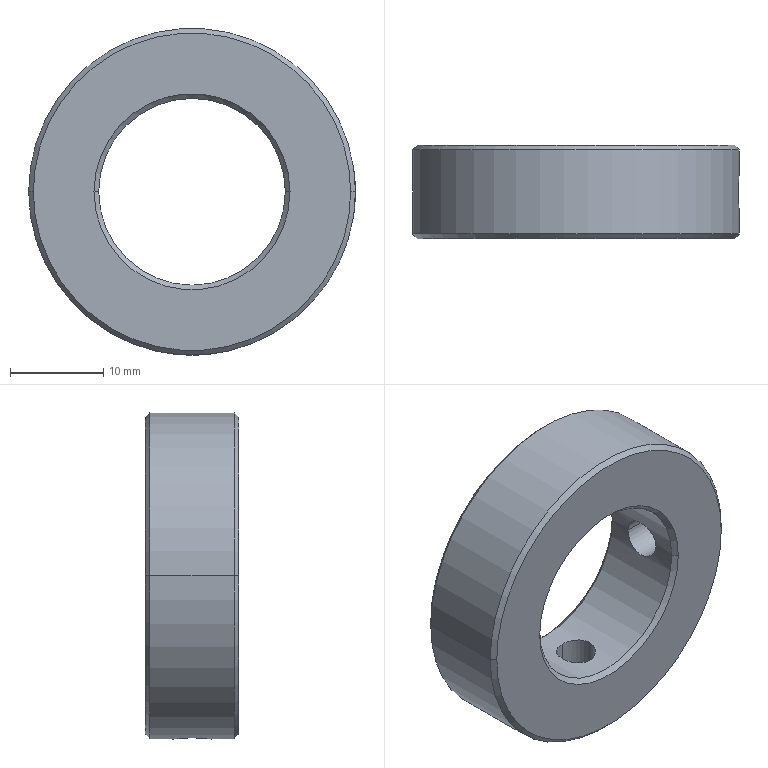Component | SolidWorks | 8TC-A15004-40-23A-1 | 1 solid | 18 faces | box 35 x 10 x 35 mm | volume 6228 mm3 | cone 8 | cylinder 8 | plane 2 | commonest cylinder face diameters 4.2 x4 20 x2 35 x2 | material A3
build123d program:
from build123d import *

# Parameters (mm, degrees)
SKETCH1_R           = 17.5
SKETCH1_R_2         = 10
BOSS_EXTRUDE1_DEPTH = 5
SKETCH2_R           = 2.1
CUT_EXTRUDE1_DEPTH  = 20
CIRPATTERN1_COUNT   = 2
CIRPATTERN1_ANGLE   = 90
CHAMFER1_SIZE       = 0.5


with BuildPart() as part:
    # Sketch1 → Boss-Extrude1 (new, symmetric)
    with BuildSketch(Plane.XY):
        Circle(SKETCH1_R)
        Circle(SKETCH1_R_2, mode=Mode.SUBTRACT)
    extrude(amount=BOSS_EXTRUDE1_DEPTH, both=True)

    # Sketch2 → Cut-Extrude1 (cut)
    with BuildSketch(Plane(origin=(0, 0, 0), x_dir=(1, 0, 0), z_dir=(0, 1, 0))):
        with Locations(Location((0, 0, 0), (0, 0, 270))):
            Circle(SKETCH2_R)
    cut_extrude1 = extrude(amount=-CUT_EXTRUDE1_DEPTH, mode=Mode.SUBTRACT)

    # CirPattern1: Cut-Extrude1 ×2 about axis
    cirpattern1_axis = Axis((0, 0, -5), (0, 0, 1))
    for i in range(1, CIRPATTERN1_COUNT):
        add(cut_extrude1.rotate(cirpattern1_axis, i * CIRPATTERN1_ANGLE / (CIRPATTERN1_COUNT - 1)), mode=Mode.SUBTRACT)

    # Chamfer1
    chamfer1_edges = [part.edges().sort_by_distance(p)[0] for p in [
        (-17.5, 0, -5),
        (-17.5, 0, 5),
        (-10, 0, -5),
        (-10, 0, 5),
    ]]
    chamfer(chamfer1_edges, length=CHAMFER1_SIZE)


solid = part.part

# Placed as in the assembly
solid = solid.moved(Location((40, 212.5, -750), (90, 0, 0)))
STEP:
#1=COLOUR_RGB('',0.7922,0.8196,0.9333);
#2=FILL_AREA_STYLE_COLOUR('',#1);
#3=FILL_AREA_STYLE('',(#2));
#4=SURFACE_STYLE_FILL_AREA(#3);
#5=SURFACE_SIDE_STYLE('',(#4));
#6=SURFACE_STYLE_USAGE(.BOTH.,#5);
#7=PRESENTATION_STYLE_ASSIGNMENT((#6));
#8=CARTESIAN_POINT('',(0.9055,8.563,-29.528));
#9=VERTEX_POINT('',#8);
#10=CARTESIAN_POINT('',(2.244,8.563,-29.528));
#11=VERTEX_POINT('',#10);
#12=CARTESIAN_POINT('',(1.575,8.563,-29.528));
#13=DIRECTION('',(0.,1.,0.));
#14=DIRECTION('',(1.,0.,0.));
#15=AXIS2_PLACEMENT_3D('',#12,#13,#14);
#16=CIRCLE('',#15,0.6693);
#17=EDGE_CURVE('',#9,#11,#16,.T.);
#18=ORIENTED_EDGE('',*,*,#17,.F.);
#19=CARTESIAN_POINT('',(0.8858,8.543,-29.528));
#20=VERTEX_POINT('',#19);
#21=CARTESIAN_POINT('',(0.8858,8.543,-29.528));
#22=DIRECTION('',(-0.7071,-0.7071,0.));
#23=VECTOR('',#22,39.37);
#24=LINE('',#21,#23);
#25=EDGE_CURVE('',#9,#20,#24,.T.);
#26=ORIENTED_EDGE('',*,*,#25,.T.);
#27=CARTESIAN_POINT('',(2.264,8.543,-29.528));
#28=VERTEX_POINT('',#27);
#29=CARTESIAN_POINT('',(1.575,8.543,-29.528));
#30=DIRECTION('',(0.,-1.,0.));
#31=DIRECTION('',(1.,0.,0.));
#32=AXIS2_PLACEMENT_3D('',#29,#30,#31);
#33=CIRCLE('',#32,0.689);
#34=EDGE_CURVE('',#28,#20,#33,.T.);
#35=ORIENTED_EDGE('',*,*,#34,.F.);
#36=CARTESIAN_POINT('',(2.264,8.543,-29.528));
#37=DIRECTION('',(0.7071,-0.7071,0.));
#38=VECTOR('',#37,39.37);
#39=LINE('',#36,#38);
#40=EDGE_CURVE('',#11,#28,#39,.T.);
#41=ORIENTED_EDGE('',*,*,#40,.F.);
#42=EDGE_LOOP('',(#18,#26,#35,#41));
#43=FACE_OUTER_BOUND('',#42,.T.);
#44=CARTESIAN_POINT('',(1.575,8.543,-29.528));
#45=DIRECTION('',(0.,-1.,0.));
#46=DIRECTION('',(1.,0.,0.));
#47=AXIS2_PLACEMENT_3D('',#44,#45,#46);
#48=CONICAL_SURFACE('',#47,0.689,0.7854);
#49=ADVANCED_FACE('',(#43),#48,.T.);
#50=CARTESIAN_POINT('',(1.969,8.543,-29.528));
#51=VERTEX_POINT('',#50);
#52=CARTESIAN_POINT('',(1.181,8.543,-29.528));
#53=VERTEX_POINT('',#52);
#54=CARTESIAN_POINT('',(1.575,8.543,-29.528));
#55=DIRECTION('',(0.,1.,0.));
#56=DIRECTION('',(1.,0.,0.));
#57=AXIS2_PLACEMENT_3D('',#54,#55,#56);
#58=CIRCLE('',#57,0.3937);
#59=EDGE_CURVE('',#51,#53,#58,.T.);
#60=ORIENTED_EDGE('',*,*,#59,.F.);
#61=CARTESIAN_POINT('',(1.988,8.563,-29.528));
#62=VERTEX_POINT('',#61);
#63=CARTESIAN_POINT('',(1.988,8.563,-29.528));
#64=DIRECTION('',(0.7071,0.7071,0.));
#65=VECTOR('',#64,39.37);
#66=LINE('',#63,#65);
#67=EDGE_CURVE('',#51,#62,#66,.T.);
#68=ORIENTED_EDGE('',*,*,#67,.T.);
#69=CARTESIAN_POINT('',(1.161,8.563,-29.528));
#70=VERTEX_POINT('',#69);
#71=CARTESIAN_POINT('',(1.575,8.563,-29.528));
#72=DIRECTION('',(0.,-1.,0.));
#73=DIRECTION('',(1.,0.,0.));
#74=AXIS2_PLACEMENT_3D('',#71,#72,#73);
#75=CIRCLE('',#74,0.4134);
#76=EDGE_CURVE('',#70,#62,#75,.T.);
#77=ORIENTED_EDGE('',*,*,#76,.F.);
#78=CARTESIAN_POINT('',(1.161,8.563,-29.528));
#79=DIRECTION('',(-0.7071,0.7071,0.));
#80=VECTOR('',#79,39.37);
#81=LINE('',#78,#80);
#82=EDGE_CURVE('',#53,#70,#81,.T.);
#83=ORIENTED_EDGE('',*,*,#82,.F.);
#84=EDGE_LOOP('',(#60,#68,#77,#83));
#85=FACE_OUTER_BOUND('',#84,.T.);
#86=CARTESIAN_POINT('',(1.575,8.563,-29.528));
#87=DIRECTION('',(0.,1.,0.));
#88=DIRECTION('',(-1.,0.,0.));
#89=AXIS2_PLACEMENT_3D('',#86,#87,#88);
#90=CONICAL_SURFACE('',#89,0.4134,0.7854);
#91=ADVANCED_FACE('',(#85),#90,.F.);
#92=CARTESIAN_POINT('',(2.244,8.169,-29.528));
#93=VERTEX_POINT('',#92);
#94=CARTESIAN_POINT('',(0.9055,8.169,-29.528));
#95=VERTEX_POINT('',#94);
#96=CARTESIAN_POINT('',(1.575,8.169,-29.528));
#97=DIRECTION('',(0.,-1.,0.));
#98=DIRECTION('',(1.,0.,0.));
#99=AXIS2_PLACEMENT_3D('',#96,#97,#98);
#100=CIRCLE('',#99,0.6693);
#101=EDGE_CURVE('',#93,#95,#100,.T.);
#102=ORIENTED_EDGE('',*,*,#101,.F.);
#103=CARTESIAN_POINT('',(2.264,8.189,-29.528));
#104=VERTEX_POINT('',#103);
#105=CARTESIAN_POINT('',(2.244,8.169,-29.528));
#106=DIRECTION('',(0.7071,0.7071,0.));
#107=VECTOR('',#106,39.37);
#108=LINE('',#105,#107);
#109=EDGE_CURVE('',#93,#104,#108,.T.);
#110=ORIENTED_EDGE('',*,*,#109,.T.);
#111=CARTESIAN_POINT('',(0.8858,8.189,-29.528));
#112=VERTEX_POINT('',#111);
#113=CARTESIAN_POINT('',(1.575,8.189,-29.528));
#114=DIRECTION('',(0.,1.,0.));
#115=DIRECTION('',(1.,0.,0.));
#116=AXIS2_PLACEMENT_3D('',#113,#114,#115);
#117=CIRCLE('',#116,0.689);
#118=EDGE_CURVE('',#112,#104,#117,.T.);
#119=ORIENTED_EDGE('',*,*,#118,.F.);
#120=CARTESIAN_POINT('',(0.9055,8.169,-29.528));
#121=DIRECTION('',(-0.7071,0.7071,0.));
#122=VECTOR('',#121,39.37);
#123=LINE('',#120,#122);
#124=EDGE_CURVE('',#95,#112,#123,.T.);
#125=ORIENTED_EDGE('',*,*,#124,.F.);
#126=EDGE_LOOP('',(#102,#110,#119,#125));
#127=FACE_OUTER_BOUND('',#126,.T.);
#128=CARTESIAN_POINT('',(1.575,8.169,-29.528));
#129=DIRECTION('',(0.,1.,0.));
#130=DIRECTION('',(-1.,0.,0.));
#131=AXIS2_PLACEMENT_3D('',#128,#129,#130);
#132=CONICAL_SURFACE('',#131,0.6693,0.7854);
#133=ADVANCED_FACE('',(#127),#132,.T.);
#134=CARTESIAN_POINT('',(1.181,8.189,-29.528));
#135=VERTEX_POINT('',#134);
#136=CARTESIAN_POINT('',(1.969,8.189,-29.528));
#137=VERTEX_POINT('',#136);
#138=CARTESIAN_POINT('',(1.575,8.189,-29.528));
#139=DIRECTION('',(0.,-1.,0.));
#140=DIRECTION('',(1.,0.,0.));
#141=AXIS2_PLACEMENT_3D('',#138,#139,#140);
#142=CIRCLE('',#141,0.3937);
#143=EDGE_CURVE('',#135,#137,#142,.T.);
#144=ORIENTED_EDGE('',*,*,#143,.F.);
#145=CARTESIAN_POINT('',(1.161,8.169,-29.528));
#146=VERTEX_POINT('',#145);
#147=CARTESIAN_POINT('',(1.181,8.189,-29.528));
#148=DIRECTION('',(-0.7071,-0.7071,0.));
#149=VECTOR('',#148,39.37);
#150=LINE('',#147,#149);
#151=EDGE_CURVE('',#135,#146,#150,.T.);
#152=ORIENTED_EDGE('',*,*,#151,.T.);
#153=CARTESIAN_POINT('',(1.988,8.169,-29.528));
#154=VERTEX_POINT('',#153);
#155=CARTESIAN_POINT('',(1.575,8.169,-29.528));
#156=DIRECTION('',(0.,1.,0.));
#157=DIRECTION('',(1.,0.,0.));
#158=AXIS2_PLACEMENT_3D('',#155,#156,#157);
#159=CIRCLE('',#158,0.4134);
#160=EDGE_CURVE('',#154,#146,#159,.T.);
#161=ORIENTED_EDGE('',*,*,#160,.F.);
#162=CARTESIAN_POINT('',(1.969,8.189,-29.528));
#163=DIRECTION('',(0.7071,-0.7071,0.));
#164=VECTOR('',#163,39.37);
#165=LINE('',#162,#164);
#166=EDGE_CURVE('',#137,#154,#165,.T.);
#167=ORIENTED_EDGE('',*,*,#166,.F.);
#168=EDGE_LOOP('',(#144,#152,#161,#167));
#169=FACE_OUTER_BOUND('',#168,.T.);
#170=CARTESIAN_POINT('',(1.575,8.189,-29.528));
#171=DIRECTION('',(0.,-1.,0.));
#172=DIRECTION('',(1.,0.,0.));
#173=AXIS2_PLACEMENT_3D('',#170,#171,#172);
#174=CONICAL_SURFACE('',#173,0.3937,0.7854);
#175=ADVANCED_FACE('',(#169),#174,.F.);
#176=CARTESIAN_POINT('',(2.264,8.449,-29.528));
#177=VERTEX_POINT('',#176);
#178=CARTESIAN_POINT('',(2.264,8.283,-29.528));
#179=VERTEX_POINT('',#178);
#180=CARTESIAN_POINT('',(2.264,8.449,-29.528));
#181=CARTESIAN_POINT('',(2.264,8.449,-29.538));
#182=CARTESIAN_POINT('',(2.264,8.447,-29.549));
#183=CARTESIAN_POINT('',(2.263,8.438,-29.569));
#184=CARTESIAN_POINT('',(2.262,8.432,-29.578));
#185=CARTESIAN_POINT('',(2.261,8.421,-29.59));
#186=CARTESIAN_POINT('',(2.261,8.417,-29.593));
#187=CARTESIAN_POINT('',(2.26,8.408,-29.599));
#188=CARTESIAN_POINT('',(2.26,8.403,-29.602));
#189=CARTESIAN_POINT('',(2.259,8.393,-29.606));
#190=CARTESIAN_POINT('',(2.259,8.388,-29.608));
#191=CARTESIAN_POINT('',(2.259,8.377,-29.61));
#192=CARTESIAN_POINT('',(2.259,8.372,-29.61));
#193=CARTESIAN_POINT('',(2.259,8.361,-29.61));
#194=CARTESIAN_POINT('',(2.259,8.355,-29.61));
#195=CARTESIAN_POINT('',(2.259,8.345,-29.608));
#196=CARTESIAN_POINT('',(2.259,8.34,-29.606));
#197=CARTESIAN_POINT('',(2.26,8.33,-29.602));
#198=CARTESIAN_POINT('',(2.26,8.325,-29.599));
#199=CARTESIAN_POINT('',(2.261,8.316,-29.593));
#200=CARTESIAN_POINT('',(2.261,8.312,-29.59));
#201=CARTESIAN_POINT('',(2.262,8.3,-29.578));
#202=CARTESIAN_POINT('',(2.263,8.294,-29.569));
#203=CARTESIAN_POINT('',(2.264,8.286,-29.549));
#204=CARTESIAN_POINT('',(2.264,8.283,-29.538));
#205=CARTESIAN_POINT('',(2.264,8.283,-29.528));
#206=B_SPLINE_CURVE_WITH_KNOTS('',3,(#180,#181,#182,#183,#184,#185,#186,#187,#188,#189,#190,#191,#192,#193,#194,#195,#196,#197,#198,#199,#200,#201,#202,#203,#204,#205),.UNSPECIFIED.,.F.,.F.,(4,2,2,2,2,2,2,2,2,2,2,2,4),(0.006571,0.007393,0.008214,0.008625,0.009035,0.009446,0.009856,0.01027,0.01068,0.01109,0.0115,0.01232,0.01314),.UNSPECIFIED.);
#207=EDGE_CURVE('',#177,#179,#206,.T.);
#208=ORIENTED_EDGE('',*,*,#207,.F.);
#209=CARTESIAN_POINT('',(1.969,8.449,-29.528));
#210=VERTEX_POINT('',#209);
#211=CARTESIAN_POINT('',(2.362,8.449,-29.528));
#212=DIRECTION('',(-1.,0.,-0.));
#213=VECTOR('',#212,39.37);
#214=LINE('',#211,#213);
#215=EDGE_CURVE('',#177,#210,#214,.T.);
#216=ORIENTED_EDGE('',*,*,#215,.T.);
#217=CARTESIAN_POINT('',(1.969,8.283,-29.528));
#218=VERTEX_POINT('',#217);
#219=CARTESIAN_POINT('',(1.969,8.449,-29.528));
#220=CARTESIAN_POINT('',(1.969,8.449,-29.538));
#221=CARTESIAN_POINT('',(1.968,8.447,-29.549));
#222=CARTESIAN_POINT('',(1.967,8.44,-29.564));
#223=CARTESIAN_POINT('',(1.966,8.438,-29.569));
#224=CARTESIAN_POINT('',(1.965,8.432,-29.578));
#225=CARTESIAN_POINT('',(1.965,8.428,-29.582));
#226=CARTESIAN_POINT('',(1.964,8.421,-29.59));
#227=CARTESIAN_POINT('',(1.963,8.417,-29.593));
#228=CARTESIAN_POINT('',(1.962,8.408,-29.599));
#229=CARTESIAN_POINT('',(1.961,8.403,-29.602));
#230=CARTESIAN_POINT('',(1.96,8.388,-29.608));
#231=CARTESIAN_POINT('',(1.96,8.377,-29.61));
#232=CARTESIAN_POINT('',(1.96,8.361,-29.61));
#233=CARTESIAN_POINT('',(1.96,8.355,-29.61));
#234=CARTESIAN_POINT('',(1.96,8.345,-29.608));
#235=CARTESIAN_POINT('',(1.961,8.339,-29.606));
#236=CARTESIAN_POINT('',(1.961,8.329,-29.602));
#237=CARTESIAN_POINT('',(1.962,8.325,-29.599));
#238=CARTESIAN_POINT('',(1.963,8.316,-29.593));
#239=CARTESIAN_POINT('',(1.964,8.312,-29.59));
#240=CARTESIAN_POINT('',(1.965,8.3,-29.578));
#241=CARTESIAN_POINT('',(1.966,8.294,-29.569));
#242=CARTESIAN_POINT('',(1.968,8.288,-29.554));
#243=CARTESIAN_POINT('',(1.968,8.286,-29.549));
#244=CARTESIAN_POINT('',(1.968,8.284,-29.538));
#245=CARTESIAN_POINT('',(1.969,8.283,-29.533));
#246=CARTESIAN_POINT('',(1.969,8.283,-29.528));
#247=B_SPLINE_CURVE_WITH_KNOTS('',3,(#219,#220,#221,#222,#223,#224,#225,#226,#227,#228,#229,#230,#231,#232,#233,#234,#235,#236,#237,#238,#239,#240,#241,#242,#243,#244,#245,#246),.UNSPECIFIED.,.F.,.F.,(4,2,2,2,2,2,2,2,2,2,2,2,2,4),(0.006584,0.007407,0.007818,0.008229,0.008641,0.009052,0.009875,0.01029,0.0107,0.01111,0.01152,0.01234,0.01275,0.01317),.UNSPECIFIED.);
#248=EDGE_CURVE('',#210,#218,#247,.T.);
#249=ORIENTED_EDGE('',*,*,#248,.T.);
#250=CARTESIAN_POINT('',(2.362,8.283,-29.528));
#251=DIRECTION('',(-1.,0.,-0.));
#252=VECTOR('',#251,39.37);
#253=LINE('',#250,#252);
#254=EDGE_CURVE('',#179,#218,#253,.T.);
#255=ORIENTED_EDGE('',*,*,#254,.F.);
#256=EDGE_LOOP('',(#208,#216,#249,#255));
#257=FACE_OUTER_BOUND('',#256,.T.);
#258=CARTESIAN_POINT('',(2.362,8.366,-29.528));
#259=DIRECTION('',(-1.,0.,-0.));
#260=DIRECTION('',(0.,-1.,0.));
#261=AXIS2_PLACEMENT_3D('',#258,#259,#260);
#262=CYLINDRICAL_SURFACE('',#261,0.08268);
#263=ADVANCED_FACE('',(#257),#262,.F.);
#264=CARTESIAN_POINT('',(1.575,8.449,-30.217));
#265=VERTEX_POINT('',#264);
#266=CARTESIAN_POINT('',(1.575,8.283,-30.217));
#267=VERTEX_POINT('',#266);
#268=CARTESIAN_POINT('',(1.575,8.449,-30.217));
#269=CARTESIAN_POINT('',(1.564,8.449,-30.217));
#270=CARTESIAN_POINT('',(1.553,8.447,-30.216));
#271=CARTESIAN_POINT('',(1.533,8.438,-30.215));
#272=CARTESIAN_POINT('',(1.524,8.432,-30.215));
#273=CARTESIAN_POINT('',(1.513,8.421,-30.214));
#274=CARTESIAN_POINT('',(1.509,8.417,-30.213));
#275=CARTESIAN_POINT('',(1.503,8.408,-30.213));
#276=CARTESIAN_POINT('',(1.501,8.403,-30.213));
#277=CARTESIAN_POINT('',(1.496,8.393,-30.212));
#278=CARTESIAN_POINT('',(1.495,8.388,-30.212));
#279=CARTESIAN_POINT('',(1.493,8.377,-30.212));
#280=CARTESIAN_POINT('',(1.492,8.372,-30.212));
#281=CARTESIAN_POINT('',(1.492,8.361,-30.212));
#282=CARTESIAN_POINT('',(1.493,8.355,-30.212));
#283=CARTESIAN_POINT('',(1.495,8.345,-30.212));
#284=CARTESIAN_POINT('',(1.496,8.34,-30.212));
#285=CARTESIAN_POINT('',(1.5,8.33,-30.213));
#286=CARTESIAN_POINT('',(1.503,8.325,-30.213));
#287=CARTESIAN_POINT('',(1.509,8.316,-30.213));
#288=CARTESIAN_POINT('',(1.512,8.312,-30.214));
#289=CARTESIAN_POINT('',(1.524,8.3,-30.215));
#290=CARTESIAN_POINT('',(1.533,8.294,-30.215));
#291=CARTESIAN_POINT('',(1.553,8.286,-30.216));
#292=CARTESIAN_POINT('',(1.564,8.283,-30.217));
#293=CARTESIAN_POINT('',(1.575,8.283,-30.217));
#294=B_SPLINE_CURVE_WITH_KNOTS('',3,(#268,#269,#270,#271,#272,#273,#274,#275,#276,#277,#278,#279,#280,#281,#282,#283,#284,#285,#286,#287,#288,#289,#290,#291,#292,#293),.UNSPECIFIED.,.F.,.F.,(4,2,2,2,2,2,2,2,2,2,2,2,4),(0.006571,0.007393,0.008214,0.008625,0.009035,0.009446,0.009856,0.01027,0.01068,0.01109,0.0115,0.01232,0.01314),.UNSPECIFIED.);
#295=EDGE_CURVE('',#265,#267,#294,.T.);
#296=ORIENTED_EDGE('',*,*,#295,.F.);
#297=CARTESIAN_POINT('',(1.575,8.449,-29.921));
#298=VERTEX_POINT('',#297);
#299=CARTESIAN_POINT('',(1.575,8.449,-30.315));
#300=DIRECTION('',(0.,0.,1.));
#301=VECTOR('',#300,39.37);
#302=LINE('',#299,#301);
#303=EDGE_CURVE('',#265,#298,#302,.T.);
#304=ORIENTED_EDGE('',*,*,#303,.T.);
#305=CARTESIAN_POINT('',(1.575,8.283,-29.921));
#306=VERTEX_POINT('',#305);
#307=CARTESIAN_POINT('',(1.575,8.449,-29.921));
#308=CARTESIAN_POINT('',(1.564,8.449,-29.921));
#309=CARTESIAN_POINT('',(1.553,8.447,-29.921));
#310=CARTESIAN_POINT('',(1.538,8.44,-29.92));
#311=CARTESIAN_POINT('',(1.533,8.438,-29.919));
#312=CARTESIAN_POINT('',(1.524,8.432,-29.918));
#313=CARTESIAN_POINT('',(1.52,8.428,-29.917));
#314=CARTESIAN_POINT('',(1.513,8.421,-29.916));
#315=CARTESIAN_POINT('',(1.509,8.417,-29.916));
#316=CARTESIAN_POINT('',(1.503,8.408,-29.915));
#317=CARTESIAN_POINT('',(1.501,8.403,-29.914));
#318=CARTESIAN_POINT('',(1.494,8.388,-29.913));
#319=CARTESIAN_POINT('',(1.492,8.377,-29.912));
#320=CARTESIAN_POINT('',(1.492,8.361,-29.912));
#321=CARTESIAN_POINT('',(1.493,8.355,-29.913));
#322=CARTESIAN_POINT('',(1.495,8.345,-29.913));
#323=CARTESIAN_POINT('',(1.496,8.339,-29.913));
#324=CARTESIAN_POINT('',(1.5,8.329,-29.914));
#325=CARTESIAN_POINT('',(1.503,8.325,-29.915));
#326=CARTESIAN_POINT('',(1.509,8.316,-29.916));
#327=CARTESIAN_POINT('',(1.513,8.312,-29.916));
#328=CARTESIAN_POINT('',(1.524,8.3,-29.918));
#329=CARTESIAN_POINT('',(1.533,8.294,-29.919));
#330=CARTESIAN_POINT('',(1.548,8.288,-29.92));
#331=CARTESIAN_POINT('',(1.553,8.286,-29.921));
#332=CARTESIAN_POINT('',(1.564,8.284,-29.921));
#333=CARTESIAN_POINT('',(1.569,8.283,-29.921));
#334=CARTESIAN_POINT('',(1.575,8.283,-29.921));
#335=B_SPLINE_CURVE_WITH_KNOTS('',3,(#307,#308,#309,#310,#311,#312,#313,#314,#315,#316,#317,#318,#319,#320,#321,#322,#323,#324,#325,#326,#327,#328,#329,#330,#331,#332,#333,#334),.UNSPECIFIED.,.F.,.F.,(4,2,2,2,2,2,2,2,2,2,2,2,2,4),(0.006584,0.007407,0.007818,0.008229,0.008641,0.009052,0.009875,0.01029,0.0107,0.01111,0.01152,0.01234,0.01275,0.01317),.UNSPECIFIED.);
#336=EDGE_CURVE('',#298,#306,#335,.T.);
#337=ORIENTED_EDGE('',*,*,#336,.T.);
#338=CARTESIAN_POINT('',(1.575,8.283,-30.315));
#339=DIRECTION('',(0.,0.,1.));
#340=VECTOR('',#339,39.37);
#341=LINE('',#338,#340);
#342=EDGE_CURVE('',#267,#306,#341,.T.);
#343=ORIENTED_EDGE('',*,*,#342,.F.);
#344=EDGE_LOOP('',(#296,#304,#337,#343));
#345=FACE_OUTER_BOUND('',#344,.T.);
#346=CARTESIAN_POINT('',(1.575,8.366,-30.315));
#347=DIRECTION('',(0.,0.,1.));
#348=DIRECTION('',(0.,-1.,0.));
#349=AXIS2_PLACEMENT_3D('',#346,#347,#348);
#350=CYLINDRICAL_SURFACE('',#349,0.08268);
#351=ADVANCED_FACE('',(#345),#350,.F.);
#352=CARTESIAN_POINT('',(1.575,8.283,-29.921));
#353=CARTESIAN_POINT('',(1.58,8.283,-29.921));
#354=CARTESIAN_POINT('',(1.586,8.284,-29.921));
#355=CARTESIAN_POINT('',(1.596,8.286,-29.921));
#356=CARTESIAN_POINT('',(1.602,8.288,-29.92));
#357=CARTESIAN_POINT('',(1.612,8.292,-29.92));
#358=CARTESIAN_POINT('',(1.616,8.294,-29.919));
#359=CARTESIAN_POINT('',(1.625,8.3,-29.918));
#360=CARTESIAN_POINT('',(1.629,8.304,-29.917));
#361=CARTESIAN_POINT('',(1.641,8.315,-29.916));
#362=CARTESIAN_POINT('',(1.647,8.325,-29.915));
#363=CARTESIAN_POINT('',(1.653,8.339,-29.913));
#364=CARTESIAN_POINT('',(1.655,8.345,-29.913));
#365=CARTESIAN_POINT('',(1.657,8.355,-29.913));
#366=CARTESIAN_POINT('',(1.657,8.361,-29.912));
#367=CARTESIAN_POINT('',(1.657,8.372,-29.912));
#368=CARTESIAN_POINT('',(1.657,8.377,-29.913));
#369=CARTESIAN_POINT('',(1.655,8.388,-29.913));
#370=CARTESIAN_POINT('',(1.653,8.393,-29.913));
#371=CARTESIAN_POINT('',(1.647,8.408,-29.915));
#372=CARTESIAN_POINT('',(1.641,8.417,-29.916));
#373=CARTESIAN_POINT('',(1.629,8.428,-29.917));
#374=CARTESIAN_POINT('',(1.625,8.432,-29.918));
#375=CARTESIAN_POINT('',(1.616,8.438,-29.919));
#376=CARTESIAN_POINT('',(1.611,8.44,-29.92));
#377=CARTESIAN_POINT('',(1.601,8.445,-29.92));
#378=CARTESIAN_POINT('',(1.596,8.446,-29.921));
#379=CARTESIAN_POINT('',(1.586,8.448,-29.921));
#380=CARTESIAN_POINT('',(1.58,8.449,-29.921));
#381=CARTESIAN_POINT('',(1.575,8.449,-29.921));
#382=B_SPLINE_CURVE_WITH_KNOTS('',3,(#352,#353,#354,#355,#356,#357,#358,#359,#360,#361,#362,#363,#364,#365,#366,#367,#368,#369,#370,#371,#372,#373,#374,#375,#376,#377,#378,#379,#380,#381),.UNSPECIFIED.,.F.,.F.,(4,2,2,2,2,2,2,2,2,2,2,2,2,2,4),(0.,0.0004115,0.000823,0.001234,0.001646,0.002469,0.00288,0.003292,0.003703,0.004115,0.004938,0.005349,0.005761,0.006172,0.006584),.UNSPECIFIED.);
#383=EDGE_CURVE('',#306,#298,#382,.T.);
#384=ORIENTED_EDGE('',*,*,#383,.F.);
#385=ORIENTED_EDGE('',*,*,#336,.F.);
#386=EDGE_LOOP('',(#384,#385));
#387=FACE_BOUND('',#386,.T.);
#388=ORIENTED_EDGE('',*,*,#143,.T.);
#389=CARTESIAN_POINT('',(1.969,8.169,-29.528));
#390=DIRECTION('',(0.,1.,0.));
#391=VECTOR('',#390,39.37);
#392=LINE('',#389,#391);
#393=EDGE_CURVE('',#137,#218,#392,.T.);
#394=ORIENTED_EDGE('',*,*,#393,.T.);
#395=ORIENTED_EDGE('',*,*,#248,.F.);
#396=CARTESIAN_POINT('',(1.969,8.169,-29.528));
#397=DIRECTION('',(0.,1.,0.));
#398=VECTOR('',#397,39.37);
#399=LINE('',#396,#398);
#400=EDGE_CURVE('',#210,#51,#399,.T.);
#401=ORIENTED_EDGE('',*,*,#400,.T.);
#402=ORIENTED_EDGE('',*,*,#59,.T.);
#403=CARTESIAN_POINT('',(1.181,8.169,-29.528));
#404=DIRECTION('',(0.,1.,0.));
#405=VECTOR('',#404,39.37);
#406=LINE('',#403,#405);
#407=EDGE_CURVE('',#135,#53,#406,.T.);
#408=ORIENTED_EDGE('',*,*,#407,.F.);
#409=EDGE_LOOP('',(#388,#394,#395,#401,#402,#408));
#410=FACE_OUTER_BOUND('',#409,.T.);
#411=CARTESIAN_POINT('',(1.575,8.169,-29.528));
#412=DIRECTION('',(0.,1.,0.));
#413=DIRECTION('',(-1.,0.,0.));
#414=AXIS2_PLACEMENT_3D('',#411,#412,#413);
#415=CYLINDRICAL_SURFACE('',#414,0.3937);
#416=ADVANCED_FACE('',(#387,#410),#415,.F.);
#417=ORIENTED_EDGE('',*,*,#118,.T.);
#418=CARTESIAN_POINT('',(2.264,8.169,-29.528));
#419=DIRECTION('',(0.,1.,0.));
#420=VECTOR('',#419,39.37);
#421=LINE('',#418,#420);
#422=EDGE_CURVE('',#104,#179,#421,.T.);
#423=ORIENTED_EDGE('',*,*,#422,.T.);
#424=CARTESIAN_POINT('',(2.264,8.283,-29.528));
#425=CARTESIAN_POINT('',(2.264,8.283,-29.522));
#426=CARTESIAN_POINT('',(2.264,8.284,-29.517));
#427=CARTESIAN_POINT('',(2.263,8.286,-29.506));
#428=CARTESIAN_POINT('',(2.263,8.288,-29.501));
#429=CARTESIAN_POINT('',(2.263,8.292,-29.491));
#430=CARTESIAN_POINT('',(2.263,8.294,-29.486));
#431=CARTESIAN_POINT('',(2.262,8.3,-29.477));
#432=CARTESIAN_POINT('',(2.262,8.304,-29.473));
#433=CARTESIAN_POINT('',(2.261,8.315,-29.461));
#434=CARTESIAN_POINT('',(2.26,8.325,-29.455));
#435=CARTESIAN_POINT('',(2.259,8.344,-29.447));
#436=CARTESIAN_POINT('',(2.259,8.355,-29.445));
#437=CARTESIAN_POINT('',(2.259,8.372,-29.445));
#438=CARTESIAN_POINT('',(2.259,8.377,-29.445));
#439=CARTESIAN_POINT('',(2.259,8.388,-29.448));
#440=CARTESIAN_POINT('',(2.259,8.393,-29.449));
#441=CARTESIAN_POINT('',(2.26,8.403,-29.453));
#442=CARTESIAN_POINT('',(2.26,8.408,-29.456));
#443=CARTESIAN_POINT('',(2.261,8.417,-29.462));
#444=CARTESIAN_POINT('',(2.261,8.421,-29.465));
#445=CARTESIAN_POINT('',(2.262,8.428,-29.473));
#446=CARTESIAN_POINT('',(2.262,8.432,-29.477));
#447=CARTESIAN_POINT('',(2.263,8.438,-29.486));
#448=CARTESIAN_POINT('',(2.263,8.44,-29.491));
#449=CARTESIAN_POINT('',(2.263,8.445,-29.501));
#450=CARTESIAN_POINT('',(2.263,8.446,-29.506));
#451=CARTESIAN_POINT('',(2.264,8.448,-29.517));
#452=CARTESIAN_POINT('',(2.264,8.449,-29.522));
#453=CARTESIAN_POINT('',(2.264,8.449,-29.528));
#454=B_SPLINE_CURVE_WITH_KNOTS('',3,(#424,#425,#426,#427,#428,#429,#430,#431,#432,#433,#434,#435,#436,#437,#438,#439,#440,#441,#442,#443,#444,#445,#446,#447,#448,#449,#450,#451,#452,#453),.UNSPECIFIED.,.F.,.F.,(4,2,2,2,2,2,2,2,2,2,2,2,2,2,4),(0.,0.0004107,0.0008214,0.001232,0.001643,0.002464,0.003286,0.003696,0.004107,0.004518,0.004929,0.005339,0.00575,0.006161,0.006571),.UNSPECIFIED.);
#455=EDGE_CURVE('',#179,#177,#454,.T.);
#456=ORIENTED_EDGE('',*,*,#455,.T.);
#457=CARTESIAN_POINT('',(2.264,8.169,-29.528));
#458=DIRECTION('',(0.,1.,0.));
#459=VECTOR('',#458,39.37);
#460=LINE('',#457,#459);
#461=EDGE_CURVE('',#177,#28,#460,.T.);
#462=ORIENTED_EDGE('',*,*,#461,.T.);
#463=ORIENTED_EDGE('',*,*,#34,.T.);
#464=CARTESIAN_POINT('',(0.8858,8.169,-29.528));
#465=DIRECTION('',(0.,1.,0.));
#466=VECTOR('',#465,39.37);
#467=LINE('',#464,#466);
#468=EDGE_CURVE('',#112,#20,#467,.T.);
#469=ORIENTED_EDGE('',*,*,#468,.F.);
#470=EDGE_LOOP('',(#417,#423,#456,#462,#463,#469));
#471=FACE_OUTER_BOUND('',#470,.T.);
#472=CARTESIAN_POINT('',(1.575,8.169,-29.528));
#473=DIRECTION('',(0.,1.,0.));
#474=DIRECTION('',(-1.,0.,0.));
#475=AXIS2_PLACEMENT_3D('',#472,#473,#474);
#476=CYLINDRICAL_SURFACE('',#475,0.689);
#477=ADVANCED_FACE('',(#471),#476,.T.);
#478=ORIENTED_EDGE('',*,*,#160,.T.);
#479=CARTESIAN_POINT('',(1.575,8.169,-29.528));
#480=DIRECTION('',(0.,1.,0.));
#481=DIRECTION('',(1.,0.,0.));
#482=AXIS2_PLACEMENT_3D('',#479,#480,#481);
#483=CIRCLE('',#482,0.4134);
#484=EDGE_CURVE('',#146,#154,#483,.T.);
#485=ORIENTED_EDGE('',*,*,#484,.T.);
#486=EDGE_LOOP('',(#478,#485));
#487=FACE_BOUND('',#486,.T.);
#488=CARTESIAN_POINT('',(1.575,8.169,-29.528));
#489=DIRECTION('',(0.,-1.,0.));
#490=DIRECTION('',(1.,0.,0.));
#491=AXIS2_PLACEMENT_3D('',#488,#489,#490);
#492=CIRCLE('',#491,0.6693);
#493=EDGE_CURVE('',#95,#93,#492,.T.);
#494=ORIENTED_EDGE('',*,*,#493,.T.);
#495=ORIENTED_EDGE('',*,*,#101,.T.);
#496=EDGE_LOOP('',(#494,#495));
#497=FACE_OUTER_BOUND('',#496,.T.);
#498=CARTESIAN_POINT('',(1.575,8.169,-29.528));
#499=DIRECTION('',(0.,-1.,0.));
#500=DIRECTION('',(1.,0.,0.));
#501=AXIS2_PLACEMENT_3D('',#498,#499,#500);
#502=PLANE('',#501);
#503=ADVANCED_FACE('',(#487,#497),#502,.T.);
#504=ORIENTED_EDGE('',*,*,#76,.T.);
#505=CARTESIAN_POINT('',(1.575,8.563,-29.528));
#506=DIRECTION('',(0.,-1.,0.));
#507=DIRECTION('',(1.,0.,0.));
#508=AXIS2_PLACEMENT_3D('',#505,#506,#507);
#509=CIRCLE('',#508,0.4134);
#510=EDGE_CURVE('',#62,#70,#509,.T.);
#511=ORIENTED_EDGE('',*,*,#510,.T.);
#512=EDGE_LOOP('',(#504,#511));
#513=FACE_BOUND('',#512,.T.);
#514=CARTESIAN_POINT('',(1.575,8.563,-29.528));
#515=DIRECTION('',(0.,1.,0.));
#516=DIRECTION('',(1.,0.,0.));
#517=AXIS2_PLACEMENT_3D('',#514,#515,#516);
#518=CIRCLE('',#517,0.6693);
#519=EDGE_CURVE('',#11,#9,#518,.T.);
#520=ORIENTED_EDGE('',*,*,#519,.T.);
#521=ORIENTED_EDGE('',*,*,#17,.T.);
#522=EDGE_LOOP('',(#520,#521));
#523=FACE_OUTER_BOUND('',#522,.T.);
#524=CARTESIAN_POINT('',(1.575,8.563,-29.528));
#525=DIRECTION('',(0.,-1.,0.));
#526=DIRECTION('',(1.,0.,0.));
#527=AXIS2_PLACEMENT_3D('',#524,#525,#526);
#528=PLANE('',#527);
#529=ADVANCED_FACE('',(#513,#523),#528,.F.);
#530=ORIENTED_EDGE('',*,*,#422,.F.);
#531=CARTESIAN_POINT('',(1.575,8.189,-29.528));
#532=DIRECTION('',(0.,1.,0.));
#533=DIRECTION('',(1.,0.,0.));
#534=AXIS2_PLACEMENT_3D('',#531,#532,#533);
#535=CIRCLE('',#534,0.689);
#536=EDGE_CURVE('',#104,#112,#535,.T.);
#537=ORIENTED_EDGE('',*,*,#536,.T.);
#538=ORIENTED_EDGE('',*,*,#468,.T.);
#539=CARTESIAN_POINT('',(1.575,8.543,-29.528));
#540=DIRECTION('',(0.,-1.,0.));
#541=DIRECTION('',(1.,0.,0.));
#542=AXIS2_PLACEMENT_3D('',#539,#540,#541);
#543=CIRCLE('',#542,0.689);
#544=EDGE_CURVE('',#20,#28,#543,.T.);
#545=ORIENTED_EDGE('',*,*,#544,.T.);
#546=ORIENTED_EDGE('',*,*,#461,.F.);
#547=ORIENTED_EDGE('',*,*,#207,.T.);
#548=EDGE_LOOP('',(#530,#537,#538,#545,#546,#547));
#549=FACE_OUTER_BOUND('',#548,.T.);
#550=CARTESIAN_POINT('',(1.575,8.283,-30.217));
#551=CARTESIAN_POINT('',(1.58,8.283,-30.217));
#552=CARTESIAN_POINT('',(1.586,8.284,-30.216));
#553=CARTESIAN_POINT('',(1.596,8.286,-30.216));
#554=CARTESIAN_POINT('',(1.601,8.288,-30.216));
#555=CARTESIAN_POINT('',(1.611,8.292,-30.216));
#556=CARTESIAN_POINT('',(1.616,8.294,-30.215));
#557=CARTESIAN_POINT('',(1.625,8.3,-30.215));
#558=CARTESIAN_POINT('',(1.629,8.304,-30.214));
#559=CARTESIAN_POINT('',(1.641,8.315,-30.213));
#560=CARTESIAN_POINT('',(1.647,8.325,-30.213));
#561=CARTESIAN_POINT('',(1.655,8.344,-30.212));
#562=CARTESIAN_POINT('',(1.657,8.355,-30.212));
#563=CARTESIAN_POINT('',(1.657,8.372,-30.212));
#564=CARTESIAN_POINT('',(1.657,8.377,-30.212));
#565=CARTESIAN_POINT('',(1.655,8.388,-30.212));
#566=CARTESIAN_POINT('',(1.653,8.393,-30.212));
#567=CARTESIAN_POINT('',(1.649,8.403,-30.213));
#568=CARTESIAN_POINT('',(1.647,8.408,-30.213));
#569=CARTESIAN_POINT('',(1.641,8.417,-30.213));
#570=CARTESIAN_POINT('',(1.637,8.421,-30.214));
#571=CARTESIAN_POINT('',(1.629,8.428,-30.214));
#572=CARTESIAN_POINT('',(1.625,8.432,-30.215));
#573=CARTESIAN_POINT('',(1.616,8.438,-30.215));
#574=CARTESIAN_POINT('',(1.611,8.44,-30.216));
#575=CARTESIAN_POINT('',(1.601,8.445,-30.216));
#576=CARTESIAN_POINT('',(1.596,8.446,-30.216));
#577=CARTESIAN_POINT('',(1.586,8.448,-30.216));
#578=CARTESIAN_POINT('',(1.58,8.449,-30.217));
#579=CARTESIAN_POINT('',(1.575,8.449,-30.217));
#580=B_SPLINE_CURVE_WITH_KNOTS('',3,(#550,#551,#552,#553,#554,#555,#556,#557,#558,#559,#560,#561,#562,#563,#564,#565,#566,#567,#568,#569,#570,#571,#572,#573,#574,#575,#576,#577,#578,#579),.UNSPECIFIED.,.F.,.F.,(4,2,2,2,2,2,2,2,2,2,2,2,2,2,4),(0.,0.0004107,0.0008214,0.001232,0.001643,0.002464,0.003286,0.003696,0.004107,0.004518,0.004929,0.005339,0.00575,0.006161,0.006571),.UNSPECIFIED.);
#581=EDGE_CURVE('',#267,#265,#580,.T.);
#582=ORIENTED_EDGE('',*,*,#581,.T.);
#583=ORIENTED_EDGE('',*,*,#295,.T.);
#584=EDGE_LOOP('',(#582,#583));
#585=FACE_BOUND('',#584,.T.);
#586=CARTESIAN_POINT('',(1.575,8.169,-29.528));
#587=DIRECTION('',(0.,1.,0.));
#588=DIRECTION('',(-1.,0.,0.));
#589=AXIS2_PLACEMENT_3D('',#586,#587,#588);
#590=CYLINDRICAL_SURFACE('',#589,0.689);
#591=ADVANCED_FACE('',(#549,#585),#590,.T.);
#592=ORIENTED_EDGE('',*,*,#393,.F.);
#593=CARTESIAN_POINT('',(1.575,8.189,-29.528));
#594=DIRECTION('',(0.,-1.,0.));
#595=DIRECTION('',(1.,0.,0.));
#596=AXIS2_PLACEMENT_3D('',#593,#594,#595);
#597=CIRCLE('',#596,0.3937);
#598=EDGE_CURVE('',#137,#135,#597,.T.);
#599=ORIENTED_EDGE('',*,*,#598,.T.);
#600=ORIENTED_EDGE('',*,*,#407,.T.);
#601=CARTESIAN_POINT('',(1.575,8.543,-29.528));
#602=DIRECTION('',(0.,1.,0.));
#603=DIRECTION('',(1.,0.,0.));
#604=AXIS2_PLACEMENT_3D('',#601,#602,#603);
#605=CIRCLE('',#604,0.3937);
#606=EDGE_CURVE('',#53,#51,#605,.T.);
#607=ORIENTED_EDGE('',*,*,#606,.T.);
#608=ORIENTED_EDGE('',*,*,#400,.F.);
#609=CARTESIAN_POINT('',(1.969,8.283,-29.528));
#610=CARTESIAN_POINT('',(1.969,8.283,-29.522));
#611=CARTESIAN_POINT('',(1.968,8.284,-29.517));
#612=CARTESIAN_POINT('',(1.968,8.286,-29.506));
#613=CARTESIAN_POINT('',(1.968,8.288,-29.501));
#614=CARTESIAN_POINT('',(1.967,8.292,-29.491));
#615=CARTESIAN_POINT('',(1.966,8.294,-29.486));
#616=CARTESIAN_POINT('',(1.965,8.3,-29.477));
#617=CARTESIAN_POINT('',(1.965,8.304,-29.473));
#618=CARTESIAN_POINT('',(1.963,8.315,-29.461));
#619=CARTESIAN_POINT('',(1.962,8.325,-29.455));
#620=CARTESIAN_POINT('',(1.961,8.339,-29.449));
#621=CARTESIAN_POINT('',(1.96,8.345,-29.448));
#622=CARTESIAN_POINT('',(1.96,8.355,-29.445));
#623=CARTESIAN_POINT('',(1.96,8.361,-29.445));
#624=CARTESIAN_POINT('',(1.96,8.372,-29.445));
#625=CARTESIAN_POINT('',(1.96,8.377,-29.445));
#626=CARTESIAN_POINT('',(1.96,8.388,-29.448));
#627=CARTESIAN_POINT('',(1.961,8.393,-29.449));
#628=CARTESIAN_POINT('',(1.962,8.408,-29.455));
#629=CARTESIAN_POINT('',(1.963,8.417,-29.461));
#630=CARTESIAN_POINT('',(1.965,8.428,-29.473));
#631=CARTESIAN_POINT('',(1.965,8.432,-29.477));
#632=CARTESIAN_POINT('',(1.966,8.438,-29.486));
#633=CARTESIAN_POINT('',(1.967,8.44,-29.491));
#634=CARTESIAN_POINT('',(1.968,8.445,-29.501));
#635=CARTESIAN_POINT('',(1.968,8.446,-29.506));
#636=CARTESIAN_POINT('',(1.968,8.448,-29.517));
#637=CARTESIAN_POINT('',(1.969,8.449,-29.522));
#638=CARTESIAN_POINT('',(1.969,8.449,-29.528));
#639=B_SPLINE_CURVE_WITH_KNOTS('',3,(#609,#610,#611,#612,#613,#614,#615,#616,#617,#618,#619,#620,#621,#622,#623,#624,#625,#626,#627,#628,#629,#630,#631,#632,#633,#634,#635,#636,#637,#638),.UNSPECIFIED.,.F.,.F.,(4,2,2,2,2,2,2,2,2,2,2,2,2,2,4),(0.,0.0004115,0.000823,0.001234,0.001646,0.002469,0.00288,0.003292,0.003703,0.004115,0.004938,0.005349,0.005761,0.006172,0.006584),.UNSPECIFIED.);
#640=EDGE_CURVE('',#218,#210,#639,.T.);
#641=ORIENTED_EDGE('',*,*,#640,.F.);
#642=EDGE_LOOP('',(#592,#599,#600,#607,#608,#641));
#643=FACE_OUTER_BOUND('',#642,.T.);
#644=CARTESIAN_POINT('',(1.575,8.169,-29.528));
#645=DIRECTION('',(0.,1.,0.));
#646=DIRECTION('',(-1.,0.,0.));
#647=AXIS2_PLACEMENT_3D('',#644,#645,#646);
#648=CYLINDRICAL_SURFACE('',#647,0.3937);
#649=ADVANCED_FACE('',(#643),#648,.F.);
#650=ORIENTED_EDGE('',*,*,#303,.F.);
#651=ORIENTED_EDGE('',*,*,#581,.F.);
#652=ORIENTED_EDGE('',*,*,#342,.T.);
#653=ORIENTED_EDGE('',*,*,#383,.T.);
#654=EDGE_LOOP('',(#650,#651,#652,#653));
#655=FACE_OUTER_BOUND('',#654,.T.);
#656=CARTESIAN_POINT('',(1.575,8.366,-30.315));
#657=DIRECTION('',(0.,0.,1.));
#658=DIRECTION('',(0.,-1.,0.));
#659=AXIS2_PLACEMENT_3D('',#656,#657,#658);
#660=CYLINDRICAL_SURFACE('',#659,0.08268);
#661=ADVANCED_FACE('',(#655),#660,.F.);
#662=ORIENTED_EDGE('',*,*,#215,.F.);
#663=ORIENTED_EDGE('',*,*,#455,.F.);
#664=ORIENTED_EDGE('',*,*,#254,.T.);
#665=ORIENTED_EDGE('',*,*,#640,.T.);
#666=EDGE_LOOP('',(#662,#663,#664,#665));
#667=FACE_OUTER_BOUND('',#666,.T.);
#668=CARTESIAN_POINT('',(2.362,8.366,-29.528));
#669=DIRECTION('',(-1.,0.,-0.));
#670=DIRECTION('',(0.,-1.,0.));
#671=AXIS2_PLACEMENT_3D('',#668,#669,#670);
#672=CYLINDRICAL_SURFACE('',#671,0.08268);
#673=ADVANCED_FACE('',(#667),#672,.F.);
#674=ORIENTED_EDGE('',*,*,#151,.F.);
#675=ORIENTED_EDGE('',*,*,#598,.F.);
#676=ORIENTED_EDGE('',*,*,#166,.T.);
#677=ORIENTED_EDGE('',*,*,#484,.F.);
#678=EDGE_LOOP('',(#674,#675,#676,#677));
#679=FACE_OUTER_BOUND('',#678,.T.);
#680=CARTESIAN_POINT('',(1.575,8.189,-29.528));
#681=DIRECTION('',(0.,-1.,0.));
#682=DIRECTION('',(1.,0.,0.));
#683=AXIS2_PLACEMENT_3D('',#680,#681,#682);
#684=CONICAL_SURFACE('',#683,0.3937,0.7854);
#685=ADVANCED_FACE('',(#679),#684,.F.);
#686=ORIENTED_EDGE('',*,*,#109,.F.);
#687=ORIENTED_EDGE('',*,*,#493,.F.);
#688=ORIENTED_EDGE('',*,*,#124,.T.);
#689=ORIENTED_EDGE('',*,*,#536,.F.);
#690=EDGE_LOOP('',(#686,#687,#688,#689));
#691=FACE_OUTER_BOUND('',#690,.T.);
#692=CARTESIAN_POINT('',(1.575,8.169,-29.528));
#693=DIRECTION('',(0.,1.,0.));
#694=DIRECTION('',(-1.,0.,0.));
#695=AXIS2_PLACEMENT_3D('',#692,#693,#694);
#696=CONICAL_SURFACE('',#695,0.6693,0.7854);
#697=ADVANCED_FACE('',(#691),#696,.T.);
#698=ORIENTED_EDGE('',*,*,#67,.F.);
#699=ORIENTED_EDGE('',*,*,#606,.F.);
#700=ORIENTED_EDGE('',*,*,#82,.T.);
#701=ORIENTED_EDGE('',*,*,#510,.F.);
#702=EDGE_LOOP('',(#698,#699,#700,#701));
#703=FACE_OUTER_BOUND('',#702,.T.);
#704=CARTESIAN_POINT('',(1.575,8.563,-29.528));
#705=DIRECTION('',(0.,1.,0.));
#706=DIRECTION('',(-1.,0.,0.));
#707=AXIS2_PLACEMENT_3D('',#704,#705,#706);
#708=CONICAL_SURFACE('',#707,0.4134,0.7854);
#709=ADVANCED_FACE('',(#703),#708,.F.);
#710=ORIENTED_EDGE('',*,*,#25,.F.);
#711=ORIENTED_EDGE('',*,*,#519,.F.);
#712=ORIENTED_EDGE('',*,*,#40,.T.);
#713=ORIENTED_EDGE('',*,*,#544,.F.);
#714=EDGE_LOOP('',(#710,#711,#712,#713));
#715=FACE_OUTER_BOUND('',#714,.T.);
#716=CARTESIAN_POINT('',(1.575,8.543,-29.528));
#717=DIRECTION('',(0.,-1.,0.));
#718=DIRECTION('',(1.,0.,0.));
#719=AXIS2_PLACEMENT_3D('',#716,#717,#718);
#720=CONICAL_SURFACE('',#719,0.689,0.7854);
#721=ADVANCED_FACE('',(#715),#720,.T.);
#722=CLOSED_SHELL('',(#49,#91,#133,#175,#263,#351,#416,#477,#503,#529,#591,#649,#661,#673,#685,#697,#709,#721));
#723=MANIFOLD_SOLID_BREP('',#722);
#724=STYLED_ITEM('',(#7),#723);
#725=(LENGTH_UNIT()NAMED_UNIT(*)SI_UNIT($,.METRE.));
#726=LENGTH_MEASURE_WITH_UNIT(LENGTH_MEASURE(0.0254),#725);
#727=DIMENSIONAL_EXPONENTS(1.,0.,0.,0.,0.,0.,0.);
#728=(CONVERSION_BASED_UNIT('',#726)LENGTH_UNIT()NAMED_UNIT(#727));
#729=UNCERTAINTY_MEASURE_WITH_UNIT(LENGTH_MEASURE(0.00001),#728,'','');
#730=(NAMED_UNIT(*)PLANE_ANGLE_UNIT()SI_UNIT($,.RADIAN.));
#731=(NAMED_UNIT(*)SI_UNIT($,.STERADIAN.)SOLID_ANGLE_UNIT());
#732=(GEOMETRIC_REPRESENTATION_CONTEXT(3)GLOBAL_UNCERTAINTY_ASSIGNED_CONTEXT((#729))GLOBAL_UNIT_ASSIGNED_CONTEXT((#728,#730,#731))REPRESENTATION_CONTEXT('',''));
#733=MECHANICAL_DESIGN_GEOMETRIC_PRESENTATION_REPRESENTATION('',(#724),#732);
#734=PRESENTATION_LAYER_ASSIGNMENT('','',(#724));
#735=CARTESIAN_POINT('',(0.,0.,0.));
#736=DIRECTION('',(0.,0.,1.));
#737=DIRECTION('',(1.,0.,0.));
#738=AXIS2_PLACEMENT_3D('',#735,#736,#737);
#739=(LENGTH_UNIT()NAMED_UNIT(*)SI_UNIT($,.METRE.));
#740=LENGTH_MEASURE_WITH_UNIT(LENGTH_MEASURE(0.0254),#739);
#741=DIMENSIONAL_EXPONENTS(1.,0.,0.,0.,0.,0.,0.);
#742=(CONVERSION_BASED_UNIT('',#740)LENGTH_UNIT()NAMED_UNIT(#741));
#743=UNCERTAINTY_MEASURE_WITH_UNIT(LENGTH_MEASURE(0.00001),#742,'','');
#744=(NAMED_UNIT(*)PLANE_ANGLE_UNIT()SI_UNIT($,.RADIAN.));
#745=(NAMED_UNIT(*)SI_UNIT($,.STERADIAN.)SOLID_ANGLE_UNIT());
#746=(GEOMETRIC_REPRESENTATION_CONTEXT(3)GLOBAL_UNCERTAINTY_ASSIGNED_CONTEXT((#743))GLOBAL_UNIT_ASSIGNED_CONTEXT((#742,#744,#745))REPRESENTATION_CONTEXT('',''));
#747=ADVANCED_BREP_SHAPE_REPRESENTATION('',(#723,#738),#746);